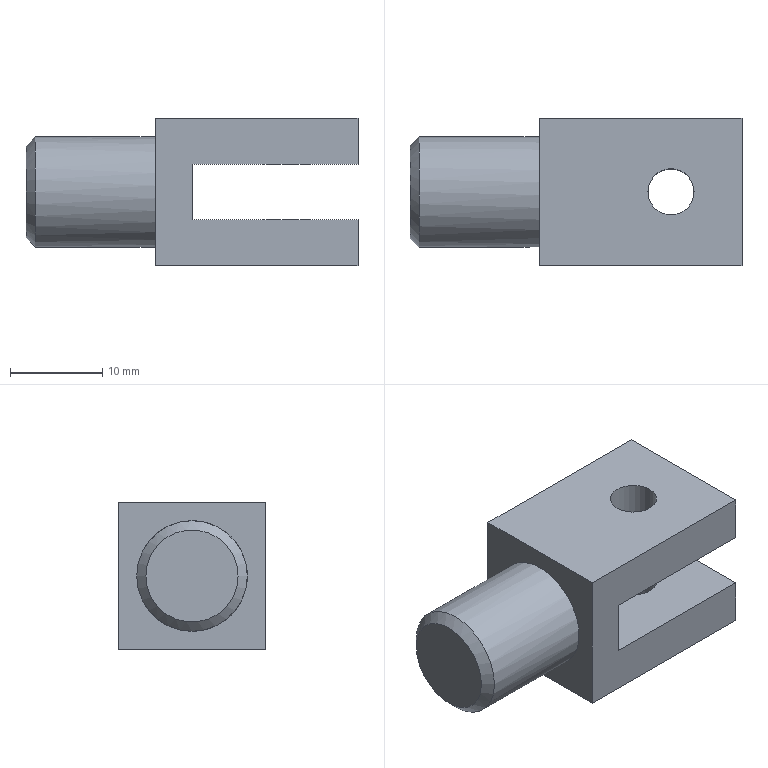Component | NX | CONNECTOR | 1 solid | 15 faces | box 36 x 16 x 16 mm | volume 5273 mm3 | plane 11 | cylinder 3 | cone 1 | commonest cylinder face diameters 5 x2 12 x1
STEP:
#1=CARTESIAN_POINT('',(0.,0.,0.));
#2=DIRECTION('',(0.,0.,1.));
#3=DIRECTION('',(1.,0.,0.));
#4=AXIS2_PLACEMENT_3D('',#1,#2,#3);
#5=CARTESIAN_POINT('',(-35.,-51.25,-19.5));
#6=VERTEX_POINT('',#5);
#7=CARTESIAN_POINT('',(-17.,-51.25,-19.5));
#8=VERTEX_POINT('',#7);
#9=CARTESIAN_POINT('',(-17.,-51.25,-19.5));
#10=DIRECTION('',(1.,0.,0.));
#11=VECTOR('',#10,1.);
#12=LINE('',#9,#11);
#13=CARTESIAN_POINT('',(-17.,-51.25,-8.5));
#14=DIRECTION('',(0.,1.,0.));
#15=DIRECTION('',(-1.,0.,0.));
#16=AXIS2_PLACEMENT_3D('',#13,#14,#15);
#17=PLANE('',#16);
#18=CARTESIAN_POINT('',(0.,-11.));
#19=DIRECTION('',(-1.,0.));
#20=VECTOR('',#19,1.);
#21=LINE('',#18,#20);
#22=(GEOMETRIC_REPRESENTATION_CONTEXT(2)PARAMETRIC_REPRESENTATION_CONTEXT()REPRESENTATION_CONTEXT('',''));
#23=DEFINITIONAL_REPRESENTATION('',(#21),#22);
#24=PCURVE('',#17,#23);
#25=CARTESIAN_POINT('',(-15.,-21.25,-19.5));
#26=DIRECTION('',(0.,0.,1.));
#27=DIRECTION('',(1.,0.,0.));
#28=AXIS2_PLACEMENT_3D('',#25,#26,#27);
#29=PLANE('',#28);
#30=CARTESIAN_POINT('',(-2.,-30.));
#31=DIRECTION('',(1.,0.));
#32=VECTOR('',#31,1.);
#33=LINE('',#30,#32);
#34=(GEOMETRIC_REPRESENTATION_CONTEXT(2)PARAMETRIC_REPRESENTATION_CONTEXT()REPRESENTATION_CONTEXT('',''));
#35=DEFINITIONAL_REPRESENTATION('',(#33),#34);
#36=PCURVE('',#29,#35);
#37=SURFACE_CURVE('',#12,(#24,#36),.PCURVE_S1.);
#38=EDGE_CURVE('',#6,#8,#37,.T.);
#39=ORIENTED_EDGE('',*,*,#38,.F.);
#40=CARTESIAN_POINT('',(-35.,-51.25,-13.5));
#41=VERTEX_POINT('',#40);
#42=CARTESIAN_POINT('',(-35.,-51.25,-8.5));
#43=DIRECTION('',(0.,0.,-1.));
#44=VECTOR('',#43,1.);
#45=LINE('',#42,#44);
#46=CARTESIAN_POINT('',(18.,0.));
#47=DIRECTION('',(0.,-1.));
#48=VECTOR('',#47,1.);
#49=LINE('',#46,#48);
#50=(GEOMETRIC_REPRESENTATION_CONTEXT(2)PARAMETRIC_REPRESENTATION_CONTEXT()REPRESENTATION_CONTEXT('',''));
#51=DEFINITIONAL_REPRESENTATION('',(#49),#50);
#52=PCURVE('',#17,#51);
#53=CARTESIAN_POINT('',(-35.,-21.25,-19.5));
#54=DIRECTION('',(1.,0.,0.));
#55=DIRECTION('',(0.,1.,0.));
#56=AXIS2_PLACEMENT_3D('',#53,#54,#55);
#57=PLANE('',#56);
#58=CARTESIAN_POINT('',(-30.,11.));
#59=DIRECTION('',(0.,-1.));
#60=VECTOR('',#59,1.);
#61=LINE('',#58,#60);
#62=(GEOMETRIC_REPRESENTATION_CONTEXT(2)PARAMETRIC_REPRESENTATION_CONTEXT()REPRESENTATION_CONTEXT('',''));
#63=DEFINITIONAL_REPRESENTATION('',(#61),#62);
#64=PCURVE('',#57,#63);
#65=SURFACE_CURVE('',#45,(#52,#64),.PCURVE_S1.);
#66=EDGE_CURVE('',#41,#6,#65,.T.);
#67=ORIENTED_EDGE('',*,*,#66,.F.);
#68=CARTESIAN_POINT('',(-17.,-51.25,-13.5));
#69=VERTEX_POINT('',#68);
#70=CARTESIAN_POINT('',(-17.,-51.25,-13.5));
#71=DIRECTION('',(-1.,0.,0.));
#72=VECTOR('',#71,1.);
#73=LINE('',#70,#72);
#74=CARTESIAN_POINT('',(0.,-5.));
#75=DIRECTION('',(1.,0.));
#76=VECTOR('',#75,1.);
#77=LINE('',#74,#76);
#78=(GEOMETRIC_REPRESENTATION_CONTEXT(2)PARAMETRIC_REPRESENTATION_CONTEXT()REPRESENTATION_CONTEXT('',''));
#79=DEFINITIONAL_REPRESENTATION('',(#77),#78);
#80=PCURVE('',#17,#79);
#81=CARTESIAN_POINT('',(-35.,-21.25,-13.5));
#82=DIRECTION('',(0.,0.,-1.));
#83=DIRECTION('',(-1.,0.,0.));
#84=AXIS2_PLACEMENT_3D('',#81,#82,#83);
#85=PLANE('',#84);
#86=CARTESIAN_POINT('',(-18.,-30.));
#87=DIRECTION('',(1.,0.));
#88=VECTOR('',#87,1.);
#89=LINE('',#86,#88);
#90=(GEOMETRIC_REPRESENTATION_CONTEXT(2)PARAMETRIC_REPRESENTATION_CONTEXT()REPRESENTATION_CONTEXT('',''));
#91=DEFINITIONAL_REPRESENTATION('',(#89),#90);
#92=PCURVE('',#85,#91);
#93=SURFACE_CURVE('',#73,(#80,#92),.PCURVE_S1.);
#94=EDGE_CURVE('',#69,#41,#93,.T.);
#95=ORIENTED_EDGE('',*,*,#94,.F.);
#96=CARTESIAN_POINT('',(-17.,-51.25,-8.5));
#97=VERTEX_POINT('',#96);
#98=CARTESIAN_POINT('',(-17.,-51.25,-8.5));
#99=DIRECTION('',(0.,0.,-1.));
#100=VECTOR('',#99,1.);
#101=LINE('',#98,#100);
#102=CARTESIAN_POINT('',(0.,0.));
#103=DIRECTION('',(0.,-1.));
#104=VECTOR('',#103,1.);
#105=LINE('',#102,#104);
#106=(GEOMETRIC_REPRESENTATION_CONTEXT(2)PARAMETRIC_REPRESENTATION_CONTEXT()REPRESENTATION_CONTEXT('',''));
#107=DEFINITIONAL_REPRESENTATION('',(#105),#106);
#108=PCURVE('',#17,#107);
#109=CARTESIAN_POINT('',(-17.,-43.25,-16.5));
#110=DIRECTION('',(1.,0.,0.));
#111=DIRECTION('',(0.,1.,0.));
#112=AXIS2_PLACEMENT_3D('',#109,#110,#111);
#113=PLANE('',#112);
#114=CARTESIAN_POINT('',(-8.,8.));
#115=DIRECTION('',(0.,-1.));
#116=VECTOR('',#115,1.);
#117=LINE('',#114,#116);
#118=(GEOMETRIC_REPRESENTATION_CONTEXT(2)PARAMETRIC_REPRESENTATION_CONTEXT()REPRESENTATION_CONTEXT('',''));
#119=DEFINITIONAL_REPRESENTATION('',(#117),#118);
#120=PCURVE('',#113,#119);
#121=SURFACE_CURVE('',#101,(#108,#120),.PCURVE_S1.);
#122=EDGE_CURVE('',#97,#69,#121,.T.);
#123=ORIENTED_EDGE('',*,*,#122,.F.);
#124=CARTESIAN_POINT('',(-39.,-51.25,-8.5));
#125=VERTEX_POINT('',#124);
#126=CARTESIAN_POINT('',(-17.,-51.25,-8.5));
#127=DIRECTION('',(-1.,0.,0.));
#128=VECTOR('',#127,1.);
#129=LINE('',#126,#128);
#130=CARTESIAN_POINT('',(0.,0.));
#131=DIRECTION('',(1.,0.));
#132=VECTOR('',#131,1.);
#133=LINE('',#130,#132);
#134=(GEOMETRIC_REPRESENTATION_CONTEXT(2)PARAMETRIC_REPRESENTATION_CONTEXT()REPRESENTATION_CONTEXT('',''));
#135=DEFINITIONAL_REPRESENTATION('',(#133),#134);
#136=PCURVE('',#17,#135);
#137=CARTESIAN_POINT('',(-17.,-35.25,-8.5));
#138=DIRECTION('',(0.,0.,-1.));
#139=DIRECTION('',(-1.,0.,0.));
#140=AXIS2_PLACEMENT_3D('',#137,#138,#139);
#141=PLANE('',#140);
#142=CARTESIAN_POINT('',(0.,-16.));
#143=DIRECTION('',(1.,0.));
#144=VECTOR('',#143,1.);
#145=LINE('',#142,#144);
#146=(GEOMETRIC_REPRESENTATION_CONTEXT(2)PARAMETRIC_REPRESENTATION_CONTEXT()REPRESENTATION_CONTEXT('',''));
#147=DEFINITIONAL_REPRESENTATION('',(#145),#146);
#148=PCURVE('',#141,#147);
#149=SURFACE_CURVE('',#129,(#136,#148),.PCURVE_S1.);
#150=EDGE_CURVE('',#97,#125,#149,.T.);
#151=ORIENTED_EDGE('',*,*,#150,.T.);
#152=CARTESIAN_POINT('',(-39.,-51.25,-24.5));
#153=VERTEX_POINT('',#152);
#154=CARTESIAN_POINT('',(-39.,-51.25,-8.5));
#155=DIRECTION('',(0.,0.,-1.));
#156=VECTOR('',#155,1.);
#157=LINE('',#154,#156);
#158=CARTESIAN_POINT('',(22.,0.));
#159=DIRECTION('',(0.,-1.));
#160=VECTOR('',#159,1.);
#161=LINE('',#158,#160);
#162=(GEOMETRIC_REPRESENTATION_CONTEXT(2)PARAMETRIC_REPRESENTATION_CONTEXT()REPRESENTATION_CONTEXT('',''));
#163=DEFINITIONAL_REPRESENTATION('',(#161),#162);
#164=PCURVE('',#17,#163);
#165=CARTESIAN_POINT('',(-39.,-43.25,-16.5));
#166=DIRECTION('',(1.,0.,0.));
#167=DIRECTION('',(0.,1.,0.));
#168=AXIS2_PLACEMENT_3D('',#165,#166,#167);
#169=PLANE('',#168);
#170=CARTESIAN_POINT('',(-8.,8.));
#171=DIRECTION('',(0.,-1.));
#172=VECTOR('',#171,1.);
#173=LINE('',#170,#172);
#174=(GEOMETRIC_REPRESENTATION_CONTEXT(2)PARAMETRIC_REPRESENTATION_CONTEXT()REPRESENTATION_CONTEXT('',''));
#175=DEFINITIONAL_REPRESENTATION('',(#173),#174);
#176=PCURVE('',#169,#175);
#177=SURFACE_CURVE('',#157,(#164,#176),.PCURVE_S1.);
#178=EDGE_CURVE('',#125,#153,#177,.T.);
#179=ORIENTED_EDGE('',*,*,#178,.T.);
#180=CARTESIAN_POINT('',(-17.,-51.25,-24.5));
#181=VERTEX_POINT('',#180);
#182=CARTESIAN_POINT('',(-17.,-51.25,-24.5));
#183=DIRECTION('',(-1.,0.,0.));
#184=VECTOR('',#183,1.);
#185=LINE('',#182,#184);
#186=CARTESIAN_POINT('',(0.,-16.));
#187=DIRECTION('',(1.,0.));
#188=VECTOR('',#187,1.);
#189=LINE('',#186,#188);
#190=(GEOMETRIC_REPRESENTATION_CONTEXT(2)PARAMETRIC_REPRESENTATION_CONTEXT()REPRESENTATION_CONTEXT('',''));
#191=DEFINITIONAL_REPRESENTATION('',(#189),#190);
#192=PCURVE('',#17,#191);
#193=CARTESIAN_POINT('',(-17.,-51.25,-24.5));
#194=DIRECTION('',(0.,0.,1.));
#195=DIRECTION('',(1.,0.,0.));
#196=AXIS2_PLACEMENT_3D('',#193,#194,#195);
#197=PLANE('',#196);
#198=CARTESIAN_POINT('',(0.,0.));
#199=DIRECTION('',(-1.,0.));
#200=VECTOR('',#199,1.);
#201=LINE('',#198,#200);
#202=(GEOMETRIC_REPRESENTATION_CONTEXT(2)PARAMETRIC_REPRESENTATION_CONTEXT()REPRESENTATION_CONTEXT('',''));
#203=DEFINITIONAL_REPRESENTATION('',(#201),#202);
#204=PCURVE('',#197,#203);
#205=SURFACE_CURVE('',#185,(#192,#204),.PCURVE_S1.);
#206=EDGE_CURVE('',#181,#153,#205,.T.);
#207=ORIENTED_EDGE('',*,*,#206,.F.);
#208=CARTESIAN_POINT('',(-17.,-51.25,-8.5));
#209=DIRECTION('',(0.,0.,-1.));
#210=VECTOR('',#209,1.);
#211=LINE('',#208,#210);
#212=CARTESIAN_POINT('',(0.,0.));
#213=DIRECTION('',(0.,-1.));
#214=VECTOR('',#213,1.);
#215=LINE('',#212,#214);
#216=(GEOMETRIC_REPRESENTATION_CONTEXT(2)PARAMETRIC_REPRESENTATION_CONTEXT()REPRESENTATION_CONTEXT('',''));
#217=DEFINITIONAL_REPRESENTATION('',(#215),#216);
#218=PCURVE('',#17,#217);
#219=CARTESIAN_POINT('',(-17.,-43.25,-16.5));
#220=DIRECTION('',(1.,0.,0.));
#221=DIRECTION('',(0.,1.,0.));
#222=AXIS2_PLACEMENT_3D('',#219,#220,#221);
#223=PLANE('',#222);
#224=CARTESIAN_POINT('',(-8.,8.));
#225=DIRECTION('',(0.,-1.));
#226=VECTOR('',#225,1.);
#227=LINE('',#224,#226);
#228=(GEOMETRIC_REPRESENTATION_CONTEXT(2)PARAMETRIC_REPRESENTATION_CONTEXT()REPRESENTATION_CONTEXT('',''));
#229=DEFINITIONAL_REPRESENTATION('',(#227),#228);
#230=PCURVE('',#223,#229);
#231=SURFACE_CURVE('',#211,(#218,#230),.PCURVE_S1.);
#232=EDGE_CURVE('',#8,#181,#231,.T.);
#233=ORIENTED_EDGE('',*,*,#232,.F.);
#234=EDGE_LOOP('',(#39,#67,#95,#123,#151,#179,#207,#233));
#235=FACE_BOUND('',#234,.T.);
#236=ADVANCED_FACE('',(#235),#17,.F.);
#237=CARTESIAN_POINT('',(-17.,-35.25,-19.5));
#238=VERTEX_POINT('',#237);
#239=CARTESIAN_POINT('',(-35.,-35.25,-19.5));
#240=VERTEX_POINT('',#239);
#241=CARTESIAN_POINT('',(-17.,-35.25,-19.5));
#242=DIRECTION('',(-1.,0.,0.));
#243=VECTOR('',#242,1.);
#244=LINE('',#241,#243);
#245=CARTESIAN_POINT('',(-17.,-35.25,-24.5));
#246=DIRECTION('',(0.,-1.,0.));
#247=DIRECTION('',(1.,0.,0.));
#248=AXIS2_PLACEMENT_3D('',#245,#246,#247);
#249=PLANE('',#248);
#250=CARTESIAN_POINT('',(0.,5.));
#251=DIRECTION('',(-1.,0.));
#252=VECTOR('',#251,1.);
#253=LINE('',#250,#252);
#254=(GEOMETRIC_REPRESENTATION_CONTEXT(2)PARAMETRIC_REPRESENTATION_CONTEXT()REPRESENTATION_CONTEXT('',''));
#255=DEFINITIONAL_REPRESENTATION('',(#253),#254);
#256=PCURVE('',#249,#255);
#257=CARTESIAN_POINT('',(-2.,-14.));
#258=DIRECTION('',(-1.,0.));
#259=VECTOR('',#258,1.);
#260=LINE('',#257,#259);
#261=(GEOMETRIC_REPRESENTATION_CONTEXT(2)PARAMETRIC_REPRESENTATION_CONTEXT()REPRESENTATION_CONTEXT('',''));
#262=DEFINITIONAL_REPRESENTATION('',(#260),#261);
#263=PCURVE('',#29,#262);
#264=SURFACE_CURVE('',#244,(#256,#263),.PCURVE_S1.);
#265=EDGE_CURVE('',#238,#240,#264,.T.);
#266=ORIENTED_EDGE('',*,*,#265,.F.);
#267=CARTESIAN_POINT('',(-17.,-35.25,-24.5));
#268=VERTEX_POINT('',#267);
#269=CARTESIAN_POINT('',(-17.,-35.25,-24.5));
#270=DIRECTION('',(0.,0.,1.));
#271=VECTOR('',#270,1.);
#272=LINE('',#269,#271);
#273=CARTESIAN_POINT('',(0.,0.));
#274=DIRECTION('',(0.,1.));
#275=VECTOR('',#274,1.);
#276=LINE('',#273,#275);
#277=(GEOMETRIC_REPRESENTATION_CONTEXT(2)PARAMETRIC_REPRESENTATION_CONTEXT()REPRESENTATION_CONTEXT('',''));
#278=DEFINITIONAL_REPRESENTATION('',(#276),#277);
#279=PCURVE('',#249,#278);
#280=CARTESIAN_POINT('',(8.,-8.));
#281=DIRECTION('',(0.,1.));
#282=VECTOR('',#281,1.);
#283=LINE('',#280,#282);
#284=(GEOMETRIC_REPRESENTATION_CONTEXT(2)PARAMETRIC_REPRESENTATION_CONTEXT()REPRESENTATION_CONTEXT('',''));
#285=DEFINITIONAL_REPRESENTATION('',(#283),#284);
#286=PCURVE('',#223,#285);
#287=SURFACE_CURVE('',#272,(#279,#286),.PCURVE_S1.);
#288=EDGE_CURVE('',#268,#238,#287,.T.);
#289=ORIENTED_EDGE('',*,*,#288,.F.);
#290=CARTESIAN_POINT('',(-39.,-35.25,-24.5));
#291=VERTEX_POINT('',#290);
#292=CARTESIAN_POINT('',(-17.,-35.25,-24.5));
#293=DIRECTION('',(-1.,0.,0.));
#294=VECTOR('',#293,1.);
#295=LINE('',#292,#294);
#296=CARTESIAN_POINT('',(0.,0.));
#297=DIRECTION('',(-1.,0.));
#298=VECTOR('',#297,1.);
#299=LINE('',#296,#298);
#300=(GEOMETRIC_REPRESENTATION_CONTEXT(2)PARAMETRIC_REPRESENTATION_CONTEXT()REPRESENTATION_CONTEXT('',''));
#301=DEFINITIONAL_REPRESENTATION('',(#299),#300);
#302=PCURVE('',#249,#301);
#303=CARTESIAN_POINT('',(0.,16.));
#304=DIRECTION('',(-1.,0.));
#305=VECTOR('',#304,1.);
#306=LINE('',#303,#305);
#307=(GEOMETRIC_REPRESENTATION_CONTEXT(2)PARAMETRIC_REPRESENTATION_CONTEXT()REPRESENTATION_CONTEXT('',''));
#308=DEFINITIONAL_REPRESENTATION('',(#306),#307);
#309=PCURVE('',#197,#308);
#310=SURFACE_CURVE('',#295,(#302,#309),.PCURVE_S1.);
#311=EDGE_CURVE('',#268,#291,#310,.T.);
#312=ORIENTED_EDGE('',*,*,#311,.T.);
#313=CARTESIAN_POINT('',(-39.,-35.25,-8.5));
#314=VERTEX_POINT('',#313);
#315=CARTESIAN_POINT('',(-39.,-35.25,-24.5));
#316=DIRECTION('',(0.,0.,1.));
#317=VECTOR('',#316,1.);
#318=LINE('',#315,#317);
#319=CARTESIAN_POINT('',(-22.,0.));
#320=DIRECTION('',(0.,1.));
#321=VECTOR('',#320,1.);
#322=LINE('',#319,#321);
#323=(GEOMETRIC_REPRESENTATION_CONTEXT(2)PARAMETRIC_REPRESENTATION_CONTEXT()REPRESENTATION_CONTEXT('',''));
#324=DEFINITIONAL_REPRESENTATION('',(#322),#323);
#325=PCURVE('',#249,#324);
#326=CARTESIAN_POINT('',(8.,-8.));
#327=DIRECTION('',(0.,1.));
#328=VECTOR('',#327,1.);
#329=LINE('',#326,#328);
#330=(GEOMETRIC_REPRESENTATION_CONTEXT(2)PARAMETRIC_REPRESENTATION_CONTEXT()REPRESENTATION_CONTEXT('',''));
#331=DEFINITIONAL_REPRESENTATION('',(#329),#330);
#332=PCURVE('',#169,#331);
#333=SURFACE_CURVE('',#318,(#325,#332),.PCURVE_S1.);
#334=EDGE_CURVE('',#291,#314,#333,.T.);
#335=ORIENTED_EDGE('',*,*,#334,.T.);
#336=CARTESIAN_POINT('',(-17.,-35.25,-8.5));
#337=VERTEX_POINT('',#336);
#338=CARTESIAN_POINT('',(-17.,-35.25,-8.5));
#339=DIRECTION('',(-1.,0.,0.));
#340=VECTOR('',#339,1.);
#341=LINE('',#338,#340);
#342=CARTESIAN_POINT('',(0.,16.));
#343=DIRECTION('',(-1.,0.));
#344=VECTOR('',#343,1.);
#345=LINE('',#342,#344);
#346=(GEOMETRIC_REPRESENTATION_CONTEXT(2)PARAMETRIC_REPRESENTATION_CONTEXT()REPRESENTATION_CONTEXT('',''));
#347=DEFINITIONAL_REPRESENTATION('',(#345),#346);
#348=PCURVE('',#249,#347);
#349=CARTESIAN_POINT('',(0.,0.));
#350=DIRECTION('',(1.,0.));
#351=VECTOR('',#350,1.);
#352=LINE('',#349,#351);
#353=(GEOMETRIC_REPRESENTATION_CONTEXT(2)PARAMETRIC_REPRESENTATION_CONTEXT()REPRESENTATION_CONTEXT('',''));
#354=DEFINITIONAL_REPRESENTATION('',(#352),#353);
#355=PCURVE('',#141,#354);
#356=SURFACE_CURVE('',#341,(#348,#355),.PCURVE_S1.);
#357=EDGE_CURVE('',#337,#314,#356,.T.);
#358=ORIENTED_EDGE('',*,*,#357,.F.);
#359=CARTESIAN_POINT('',(-17.,-35.25,-13.5));
#360=VERTEX_POINT('',#359);
#361=CARTESIAN_POINT('',(-17.,-35.25,-24.5));
#362=DIRECTION('',(0.,0.,1.));
#363=VECTOR('',#362,1.);
#364=LINE('',#361,#363);
#365=CARTESIAN_POINT('',(0.,0.));
#366=DIRECTION('',(0.,1.));
#367=VECTOR('',#366,1.);
#368=LINE('',#365,#367);
#369=(GEOMETRIC_REPRESENTATION_CONTEXT(2)PARAMETRIC_REPRESENTATION_CONTEXT()REPRESENTATION_CONTEXT('',''));
#370=DEFINITIONAL_REPRESENTATION('',(#368),#369);
#371=PCURVE('',#249,#370);
#372=CARTESIAN_POINT('',(8.,-8.));
#373=DIRECTION('',(0.,1.));
#374=VECTOR('',#373,1.);
#375=LINE('',#372,#374);
#376=(GEOMETRIC_REPRESENTATION_CONTEXT(2)PARAMETRIC_REPRESENTATION_CONTEXT()REPRESENTATION_CONTEXT('',''));
#377=DEFINITIONAL_REPRESENTATION('',(#375),#376);
#378=PCURVE('',#113,#377);
#379=SURFACE_CURVE('',#364,(#371,#378),.PCURVE_S1.);
#380=EDGE_CURVE('',#360,#337,#379,.T.);
#381=ORIENTED_EDGE('',*,*,#380,.F.);
#382=CARTESIAN_POINT('',(-35.,-35.25,-13.5));
#383=VERTEX_POINT('',#382);
#384=CARTESIAN_POINT('',(-17.,-35.25,-13.5));
#385=DIRECTION('',(1.,0.,0.));
#386=VECTOR('',#385,1.);
#387=LINE('',#384,#386);
#388=CARTESIAN_POINT('',(0.,11.));
#389=DIRECTION('',(1.,0.));
#390=VECTOR('',#389,1.);
#391=LINE('',#388,#390);
#392=(GEOMETRIC_REPRESENTATION_CONTEXT(2)PARAMETRIC_REPRESENTATION_CONTEXT()REPRESENTATION_CONTEXT('',''));
#393=DEFINITIONAL_REPRESENTATION('',(#391),#392);
#394=PCURVE('',#249,#393);
#395=CARTESIAN_POINT('',(-18.,-14.));
#396=DIRECTION('',(-1.,0.));
#397=VECTOR('',#396,1.);
#398=LINE('',#395,#397);
#399=(GEOMETRIC_REPRESENTATION_CONTEXT(2)PARAMETRIC_REPRESENTATION_CONTEXT()REPRESENTATION_CONTEXT('',''));
#400=DEFINITIONAL_REPRESENTATION('',(#398),#399);
#401=PCURVE('',#85,#400);
#402=SURFACE_CURVE('',#387,(#394,#401),.PCURVE_S1.);
#403=EDGE_CURVE('',#383,#360,#402,.T.);
#404=ORIENTED_EDGE('',*,*,#403,.F.);
#405=CARTESIAN_POINT('',(-35.,-35.25,-24.5));
#406=DIRECTION('',(0.,0.,1.));
#407=VECTOR('',#406,1.);
#408=LINE('',#405,#407);
#409=CARTESIAN_POINT('',(-18.,0.));
#410=DIRECTION('',(0.,1.));
#411=VECTOR('',#410,1.);
#412=LINE('',#409,#411);
#413=(GEOMETRIC_REPRESENTATION_CONTEXT(2)PARAMETRIC_REPRESENTATION_CONTEXT()REPRESENTATION_CONTEXT('',''));
#414=DEFINITIONAL_REPRESENTATION('',(#412),#413);
#415=PCURVE('',#249,#414);
#416=CARTESIAN_POINT('',(-14.,-5.));
#417=DIRECTION('',(0.,1.));
#418=VECTOR('',#417,1.);
#419=LINE('',#416,#418);
#420=(GEOMETRIC_REPRESENTATION_CONTEXT(2)PARAMETRIC_REPRESENTATION_CONTEXT()REPRESENTATION_CONTEXT('',''));
#421=DEFINITIONAL_REPRESENTATION('',(#419),#420);
#422=PCURVE('',#57,#421);
#423=SURFACE_CURVE('',#408,(#415,#422),.PCURVE_S1.);
#424=EDGE_CURVE('',#240,#383,#423,.T.);
#425=ORIENTED_EDGE('',*,*,#424,.F.);
#426=EDGE_LOOP('',(#266,#289,#312,#335,#358,#381,#404,#425));
#427=FACE_BOUND('',#426,.T.);
#428=ADVANCED_FACE('',(#427),#249,.F.);
#429=ORIENTED_EDGE('',*,*,#288,.T.);
#430=CARTESIAN_POINT('',(-17.,-43.25,-19.5));
#431=DIRECTION('',(0.,-1.,0.));
#432=VECTOR('',#431,1.);
#433=LINE('',#430,#432);
#434=CARTESIAN_POINT('',(0.,-3.));
#435=DIRECTION('',(-1.,0.));
#436=VECTOR('',#435,1.);
#437=LINE('',#434,#436);
#438=(GEOMETRIC_REPRESENTATION_CONTEXT(2)PARAMETRIC_REPRESENTATION_CONTEXT()REPRESENTATION_CONTEXT('',''));
#439=DEFINITIONAL_REPRESENTATION('',(#437),#438);
#440=PCURVE('',#223,#439);
#441=CARTESIAN_POINT('',(-2.,-22.));
#442=DIRECTION('',(0.,-1.));
#443=VECTOR('',#442,1.);
#444=LINE('',#441,#443);
#445=(GEOMETRIC_REPRESENTATION_CONTEXT(2)PARAMETRIC_REPRESENTATION_CONTEXT()REPRESENTATION_CONTEXT('',''));
#446=DEFINITIONAL_REPRESENTATION('',(#444),#445);
#447=PCURVE('',#29,#446);
#448=SURFACE_CURVE('',#433,(#440,#447),.PCURVE_S1.);
#449=EDGE_CURVE('',#238,#8,#448,.T.);
#450=ORIENTED_EDGE('',*,*,#449,.T.);
#451=ORIENTED_EDGE('',*,*,#232,.T.);
#452=CARTESIAN_POINT('',(-17.,-51.25,-24.5));
#453=DIRECTION('',(0.,1.,0.));
#454=VECTOR('',#453,1.);
#455=LINE('',#452,#454);
#456=CARTESIAN_POINT('',(-8.,-8.));
#457=DIRECTION('',(1.,0.));
#458=VECTOR('',#457,1.);
#459=LINE('',#456,#458);
#460=(GEOMETRIC_REPRESENTATION_CONTEXT(2)PARAMETRIC_REPRESENTATION_CONTEXT()REPRESENTATION_CONTEXT('',''));
#461=DEFINITIONAL_REPRESENTATION('',(#459),#460);
#462=PCURVE('',#223,#461);
#463=CARTESIAN_POINT('',(0.,0.));
#464=DIRECTION('',(0.,1.));
#465=VECTOR('',#464,1.);
#466=LINE('',#463,#465);
#467=(GEOMETRIC_REPRESENTATION_CONTEXT(2)PARAMETRIC_REPRESENTATION_CONTEXT()REPRESENTATION_CONTEXT('',''));
#468=DEFINITIONAL_REPRESENTATION('',(#466),#467);
#469=PCURVE('',#197,#468);
#470=SURFACE_CURVE('',#455,(#462,#469),.PCURVE_S1.);
#471=EDGE_CURVE('',#181,#268,#470,.T.);
#472=ORIENTED_EDGE('',*,*,#471,.T.);
#473=EDGE_LOOP('',(#429,#450,#451,#472));
#474=FACE_BOUND('',#473,.T.);
#475=ADVANCED_FACE('',(#474),#223,.T.);
#476=ORIENTED_EDGE('',*,*,#122,.T.);
#477=CARTESIAN_POINT('',(-17.,-43.25,-13.5));
#478=DIRECTION('',(0.,1.,0.));
#479=VECTOR('',#478,1.);
#480=LINE('',#477,#479);
#481=CARTESIAN_POINT('',(0.,3.));
#482=DIRECTION('',(1.,0.));
#483=VECTOR('',#482,1.);
#484=LINE('',#481,#483);
#485=(GEOMETRIC_REPRESENTATION_CONTEXT(2)PARAMETRIC_REPRESENTATION_CONTEXT()REPRESENTATION_CONTEXT('',''));
#486=DEFINITIONAL_REPRESENTATION('',(#484),#485);
#487=PCURVE('',#113,#486);
#488=CARTESIAN_POINT('',(-18.,-22.));
#489=DIRECTION('',(0.,1.));
#490=VECTOR('',#489,1.);
#491=LINE('',#488,#490);
#492=(GEOMETRIC_REPRESENTATION_CONTEXT(2)PARAMETRIC_REPRESENTATION_CONTEXT()REPRESENTATION_CONTEXT('',''));
#493=DEFINITIONAL_REPRESENTATION('',(#491),#492);
#494=PCURVE('',#85,#493);
#495=SURFACE_CURVE('',#480,(#487,#494),.PCURVE_S1.);
#496=EDGE_CURVE('',#69,#360,#495,.T.);
#497=ORIENTED_EDGE('',*,*,#496,.T.);
#498=ORIENTED_EDGE('',*,*,#380,.T.);
#499=CARTESIAN_POINT('',(-17.,-35.25,-8.5));
#500=DIRECTION('',(0.,-1.,0.));
#501=VECTOR('',#500,1.);
#502=LINE('',#499,#501);
#503=CARTESIAN_POINT('',(8.,8.));
#504=DIRECTION('',(-1.,0.));
#505=VECTOR('',#504,1.);
#506=LINE('',#503,#505);
#507=(GEOMETRIC_REPRESENTATION_CONTEXT(2)PARAMETRIC_REPRESENTATION_CONTEXT()REPRESENTATION_CONTEXT('',''));
#508=DEFINITIONAL_REPRESENTATION('',(#506),#507);
#509=PCURVE('',#113,#508);
#510=CARTESIAN_POINT('',(0.,0.));
#511=DIRECTION('',(0.,-1.));
#512=VECTOR('',#511,1.);
#513=LINE('',#510,#512);
#514=(GEOMETRIC_REPRESENTATION_CONTEXT(2)PARAMETRIC_REPRESENTATION_CONTEXT()REPRESENTATION_CONTEXT('',''));
#515=DEFINITIONAL_REPRESENTATION('',(#513),#514);
#516=PCURVE('',#141,#515);
#517=SURFACE_CURVE('',#502,(#509,#516),.PCURVE_S1.);
#518=EDGE_CURVE('',#337,#97,#517,.T.);
#519=ORIENTED_EDGE('',*,*,#518,.T.);
#520=EDGE_LOOP('',(#476,#497,#498,#519));
#521=FACE_BOUND('',#520,.T.);
#522=ADVANCED_FACE('',(#521),#113,.T.);
#523=CARTESIAN_POINT('',(-53.,-48.25,-16.5));
#524=VERTEX_POINT('',#523);
#525=CARTESIAN_POINT('',(-53.,-43.25,-16.5));
#526=DIRECTION('',(-1.,0.,0.));
#527=DIRECTION('',(0.,-1.,0.));
#528=AXIS2_PLACEMENT_3D('',#525,#526,#527);
#529=CIRCLE('',#528,5.);
#530=CARTESIAN_POINT('',(-53.,-43.25,-16.5));
#531=DIRECTION('',(-1.,0.,0.));
#532=DIRECTION('',(0.,-1.,0.));
#533=AXIS2_PLACEMENT_3D('',#530,#531,#532);
#534=PLANE('',#533);
#535=CARTESIAN_POINT('',(0.,0.));
#536=DIRECTION('',(1.,0.));
#537=AXIS2_PLACEMENT_2D('',#535,#536);
#538=CIRCLE('',#537,5.);
#539=(GEOMETRIC_REPRESENTATION_CONTEXT(2)PARAMETRIC_REPRESENTATION_CONTEXT()REPRESENTATION_CONTEXT('',''));
#540=DEFINITIONAL_REPRESENTATION('',(#538),#539);
#541=PCURVE('',#534,#540);
#542=CARTESIAN_POINT('',(-52.,-43.25,-16.5));
#543=DIRECTION('',(1.,0.,0.));
#544=DIRECTION('',(0.,1.,0.));
#545=AXIS2_PLACEMENT_3D('',#542,#543,#544);
#546=CONICAL_SURFACE('',#545,6.,0.7854);
#547=CARTESIAN_POINT('',(9.425,-1.));
#548=DIRECTION('',(-1.,0.));
#549=VECTOR('',#548,1.);
#550=LINE('',#547,#549);
#551=(GEOMETRIC_REPRESENTATION_CONTEXT(2)PARAMETRIC_REPRESENTATION_CONTEXT()REPRESENTATION_CONTEXT('',''));
#552=DEFINITIONAL_REPRESENTATION('',(#550),#551);
#553=PCURVE('',#546,#552);
#554=SURFACE_CURVE('',#529,(#541,#553),.PCURVE_S1.);
#555=EDGE_CURVE('',#524,#524,#554,.T.);
#556=ORIENTED_EDGE('',*,*,#555,.T.);
#557=EDGE_LOOP('',(#556));
#558=FACE_BOUND('',#557,.T.);
#559=ADVANCED_FACE('',(#558),#534,.T.);
#560=CARTESIAN_POINT('',(-52.,-49.25,-16.5));
#561=VERTEX_POINT('',#560);
#562=CARTESIAN_POINT('',(-52.,-37.25,-16.5));
#563=VERTEX_POINT('',#562);
#564=CARTESIAN_POINT('',(-52.,-43.25,-16.5));
#565=DIRECTION('',(1.,0.,0.));
#566=DIRECTION('',(0.,-1.,0.));
#567=AXIS2_PLACEMENT_3D('',#564,#565,#566);
#568=CIRCLE('',#567,6.);
#569=CARTESIAN_POINT('',(-53.,-43.25,-16.5));
#570=DIRECTION('',(1.,0.,0.));
#571=DIRECTION('',(0.,1.,0.));
#572=AXIS2_PLACEMENT_3D('',#569,#570,#571);
#573=CYLINDRICAL_SURFACE('',#572,6.);
#574=CARTESIAN_POINT('',(3.142,1.));
#575=DIRECTION('',(1.,0.));
#576=VECTOR('',#575,1.);
#577=LINE('',#574,#576);
#578=(GEOMETRIC_REPRESENTATION_CONTEXT(2)PARAMETRIC_REPRESENTATION_CONTEXT()REPRESENTATION_CONTEXT('',''));
#579=DEFINITIONAL_REPRESENTATION('',(#577),#578);
#580=PCURVE('',#573,#579);
#581=CARTESIAN_POINT('',(3.142,0.));
#582=DIRECTION('',(1.,0.));
#583=VECTOR('',#582,1.);
#584=LINE('',#581,#583);
#585=(GEOMETRIC_REPRESENTATION_CONTEXT(2)PARAMETRIC_REPRESENTATION_CONTEXT()REPRESENTATION_CONTEXT('',''));
#586=DEFINITIONAL_REPRESENTATION('',(#584),#585);
#587=PCURVE('',#546,#586);
#588=SURFACE_CURVE('',#568,(#580,#587),.PCURVE_S1.);
#589=EDGE_CURVE('',#561,#563,#588,.T.);
#590=ORIENTED_EDGE('',*,*,#589,.T.);
#591=CARTESIAN_POINT('',(-39.,-37.25,-16.5));
#592=VERTEX_POINT('',#591);
#593=CARTESIAN_POINT('',(-52.,-37.25,-16.5));
#594=CARTESIAN_POINT('',(-39.,-37.25,-16.5));
#595=B_SPLINE_CURVE_WITH_KNOTS('',1,(#593,#594),.UNSPECIFIED.,.F.,.F.,(2,2),(1.,14.),.PIECEWISE_BEZIER_KNOTS.);
#596=CARTESIAN_POINT('',(6.283,0.));
#597=DIRECTION('',(0.,1.));
#598=VECTOR('',#597,1.);
#599=LINE('',#596,#598);
#600=(GEOMETRIC_REPRESENTATION_CONTEXT(2)PARAMETRIC_REPRESENTATION_CONTEXT()REPRESENTATION_CONTEXT('',''));
#601=DEFINITIONAL_REPRESENTATION('',(#599),#600);
#602=PCURVE('',#573,#601);
#603=CARTESIAN_POINT('',(0.,0.));
#604=DIRECTION('',(0.,1.));
#605=VECTOR('',#604,1.);
#606=LINE('',#603,#605);
#607=(GEOMETRIC_REPRESENTATION_CONTEXT(2)PARAMETRIC_REPRESENTATION_CONTEXT()REPRESENTATION_CONTEXT('',''));
#608=DEFINITIONAL_REPRESENTATION('',(#606),#607);
#609=PCURVE('',#573,#608);
#610=SEAM_CURVE('',#595,(#602,#609),.PCURVE_S1.);
#611=EDGE_CURVE('',#563,#592,#610,.T.);
#612=ORIENTED_EDGE('',*,*,#611,.T.);
#613=CARTESIAN_POINT('',(-39.,-43.25,-16.5));
#614=DIRECTION('',(-1.,0.,0.));
#615=DIRECTION('',(0.,1.,0.));
#616=AXIS2_PLACEMENT_3D('',#613,#614,#615);
#617=CIRCLE('',#616,6.);
#618=CARTESIAN_POINT('',(6.283,14.));
#619=DIRECTION('',(-1.,0.));
#620=VECTOR('',#619,1.);
#621=LINE('',#618,#620);
#622=(GEOMETRIC_REPRESENTATION_CONTEXT(2)PARAMETRIC_REPRESENTATION_CONTEXT()REPRESENTATION_CONTEXT('',''));
#623=DEFINITIONAL_REPRESENTATION('',(#621),#622);
#624=PCURVE('',#573,#623);
#625=CARTESIAN_POINT('',(6.,0.));
#626=CARTESIAN_POINT('',(6.,-10.392));
#627=CARTESIAN_POINT('',(-3.,-5.196));
#628=CARTESIAN_POINT('',(-12.,-0.));
#629=CARTESIAN_POINT('',(-3.,5.196));
#630=CARTESIAN_POINT('',(6.,10.392));
#631=CARTESIAN_POINT('',(6.,0.));
#632=(BOUNDED_CURVE()B_SPLINE_CURVE(2,(#625,#626,#627,#628,#629,#630,#631),.UNSPECIFIED.,.T.,.F.)B_SPLINE_CURVE_WITH_KNOTS((1,2,2,2,2,1),(-2.094,0.,2.094,4.189,6.283,8.378),.UNSPECIFIED.)CURVE()GEOMETRIC_REPRESENTATION_ITEM()RATIONAL_B_SPLINE_CURVE((1.,0.5,1.,0.5,1.,0.5,1.))REPRESENTATION_ITEM(''));
#633=(GEOMETRIC_REPRESENTATION_CONTEXT(2)PARAMETRIC_REPRESENTATION_CONTEXT()REPRESENTATION_CONTEXT('',''));
#634=DEFINITIONAL_REPRESENTATION('',(#632),#633);
#635=PCURVE('',#169,#634);
#636=SURFACE_CURVE('',#617,(#624,#635),.PCURVE_S1.);
#637=EDGE_CURVE('',#592,#592,#636,.T.);
#638=ORIENTED_EDGE('',*,*,#637,.T.);
#639=ORIENTED_EDGE('',*,*,#611,.F.);
#640=CARTESIAN_POINT('',(-52.,-43.25,-16.5));
#641=DIRECTION('',(1.,0.,0.));
#642=DIRECTION('',(0.,-1.,0.));
#643=AXIS2_PLACEMENT_3D('',#640,#641,#642);
#644=CIRCLE('',#643,6.);
#645=CARTESIAN_POINT('',(-3.142,1.));
#646=DIRECTION('',(1.,0.));
#647=VECTOR('',#646,1.);
#648=LINE('',#645,#647);
#649=(GEOMETRIC_REPRESENTATION_CONTEXT(2)PARAMETRIC_REPRESENTATION_CONTEXT()REPRESENTATION_CONTEXT('',''));
#650=DEFINITIONAL_REPRESENTATION('',(#648),#649);
#651=PCURVE('',#573,#650);
#652=CARTESIAN_POINT('',(3.142,0.));
#653=DIRECTION('',(1.,0.));
#654=VECTOR('',#653,1.);
#655=LINE('',#652,#654);
#656=(GEOMETRIC_REPRESENTATION_CONTEXT(2)PARAMETRIC_REPRESENTATION_CONTEXT()REPRESENTATION_CONTEXT('',''));
#657=DEFINITIONAL_REPRESENTATION('',(#655),#656);
#658=PCURVE('',#546,#657);
#659=SURFACE_CURVE('',#644,(#651,#658),.PCURVE_S1.);
#660=EDGE_CURVE('',#563,#561,#659,.T.);
#661=ORIENTED_EDGE('',*,*,#660,.T.);
#662=EDGE_LOOP('',(#590,#612,#638,#639,#661));
#663=FACE_BOUND('',#662,.T.);
#664=ADVANCED_FACE('',(#663),#573,.T.);
#665=CARTESIAN_POINT('',(-22.2,-43.25,-24.5));
#666=VERTEX_POINT('',#665);
#667=CARTESIAN_POINT('',(-24.7,-43.25,-24.5));
#668=DIRECTION('',(0.,0.,-1.));
#669=DIRECTION('',(1.,0.,0.));
#670=AXIS2_PLACEMENT_3D('',#667,#668,#669);
#671=CIRCLE('',#670,2.5);
#672=CARTESIAN_POINT('',(-5.2,8.));
#673=CARTESIAN_POINT('',(-5.2,3.67));
#674=CARTESIAN_POINT('',(-8.95,5.835));
#675=CARTESIAN_POINT('',(-12.7,8.));
#676=CARTESIAN_POINT('',(-8.95,10.165));
#677=CARTESIAN_POINT('',(-5.2,12.33));
#678=CARTESIAN_POINT('',(-5.2,8.));
#679=(BOUNDED_CURVE()B_SPLINE_CURVE(2,(#672,#673,#674,#675,#676,#677,#678),.UNSPECIFIED.,.T.,.F.)B_SPLINE_CURVE_WITH_KNOTS((1,2,2,2,2,1),(-2.094,0.,2.094,4.189,6.283,8.378),.UNSPECIFIED.)CURVE()GEOMETRIC_REPRESENTATION_ITEM()RATIONAL_B_SPLINE_CURVE((1.,0.5,1.,0.5,1.,0.5,1.))REPRESENTATION_ITEM(''));
#680=(GEOMETRIC_REPRESENTATION_CONTEXT(2)PARAMETRIC_REPRESENTATION_CONTEXT()REPRESENTATION_CONTEXT('',''));
#681=DEFINITIONAL_REPRESENTATION('',(#679),#680);
#682=PCURVE('',#197,#681);
#683=CARTESIAN_POINT('',(-24.7,-43.25,-38.5));
#684=DIRECTION('',(0.,0.,1.));
#685=DIRECTION('',(1.,0.,0.));
#686=AXIS2_PLACEMENT_3D('',#683,#684,#685);
#687=CYLINDRICAL_SURFACE('',#686,2.5);
#688=CARTESIAN_POINT('',(6.283,14.));
#689=DIRECTION('',(-1.,0.));
#690=VECTOR('',#689,1.);
#691=LINE('',#688,#690);
#692=(GEOMETRIC_REPRESENTATION_CONTEXT(2)PARAMETRIC_REPRESENTATION_CONTEXT()REPRESENTATION_CONTEXT('',''));
#693=DEFINITIONAL_REPRESENTATION('',(#691),#692);
#694=PCURVE('',#687,#693);
#695=SURFACE_CURVE('',#671,(#682,#694),.PCURVE_S1.);
#696=EDGE_CURVE('',#666,#666,#695,.T.);
#697=ORIENTED_EDGE('',*,*,#696,.F.);
#698=EDGE_LOOP('',(#697));
#699=FACE_BOUND('',#698,.T.);
#700=CARTESIAN_POINT('',(-39.,-51.25,-24.5));
#701=DIRECTION('',(0.,1.,0.));
#702=VECTOR('',#701,1.);
#703=LINE('',#700,#702);
#704=CARTESIAN_POINT('',(-22.,0.));
#705=DIRECTION('',(0.,1.));
#706=VECTOR('',#705,1.);
#707=LINE('',#704,#706);
#708=(GEOMETRIC_REPRESENTATION_CONTEXT(2)PARAMETRIC_REPRESENTATION_CONTEXT()REPRESENTATION_CONTEXT('',''));
#709=DEFINITIONAL_REPRESENTATION('',(#707),#708);
#710=PCURVE('',#197,#709);
#711=CARTESIAN_POINT('',(-8.,-8.));
#712=DIRECTION('',(1.,0.));
#713=VECTOR('',#712,1.);
#714=LINE('',#711,#713);
#715=(GEOMETRIC_REPRESENTATION_CONTEXT(2)PARAMETRIC_REPRESENTATION_CONTEXT()REPRESENTATION_CONTEXT('',''));
#716=DEFINITIONAL_REPRESENTATION('',(#714),#715);
#717=PCURVE('',#169,#716);
#718=SURFACE_CURVE('',#703,(#710,#717),.PCURVE_S1.);
#719=EDGE_CURVE('',#153,#291,#718,.T.);
#720=ORIENTED_EDGE('',*,*,#719,.T.);
#721=ORIENTED_EDGE('',*,*,#311,.F.);
#722=ORIENTED_EDGE('',*,*,#471,.F.);
#723=ORIENTED_EDGE('',*,*,#206,.T.);
#724=EDGE_LOOP('',(#720,#721,#722,#723));
#725=FACE_BOUND('',#724,.T.);
#726=ADVANCED_FACE('',(#699,#725),#197,.F.);
#727=CARTESIAN_POINT('',(-27.2,-43.25,-8.5));
#728=VERTEX_POINT('',#727);
#729=CARTESIAN_POINT('',(-24.7,-43.25,-8.5));
#730=DIRECTION('',(0.,0.,1.));
#731=DIRECTION('',(-1.,0.,0.));
#732=AXIS2_PLACEMENT_3D('',#729,#730,#731);
#733=CIRCLE('',#732,2.5);
#734=CARTESIAN_POINT('',(10.2,-8.));
#735=CARTESIAN_POINT('',(10.2,-12.33));
#736=CARTESIAN_POINT('',(6.45,-10.165));
#737=CARTESIAN_POINT('',(2.7,-8.));
#738=CARTESIAN_POINT('',(6.45,-5.835));
#739=CARTESIAN_POINT('',(10.2,-3.67));
#740=CARTESIAN_POINT('',(10.2,-8.));
#741=(BOUNDED_CURVE()B_SPLINE_CURVE(2,(#734,#735,#736,#737,#738,#739,#740),.UNSPECIFIED.,.T.,.F.)B_SPLINE_CURVE_WITH_KNOTS((1,2,2,2,2,1),(-2.094,0.,2.094,4.189,6.283,8.378),.UNSPECIFIED.)CURVE()GEOMETRIC_REPRESENTATION_ITEM()RATIONAL_B_SPLINE_CURVE((1.,0.5,1.,0.5,1.,0.5,1.))REPRESENTATION_ITEM(''));
#742=(GEOMETRIC_REPRESENTATION_CONTEXT(2)PARAMETRIC_REPRESENTATION_CONTEXT()REPRESENTATION_CONTEXT('',''));
#743=DEFINITIONAL_REPRESENTATION('',(#741),#742);
#744=PCURVE('',#141,#743);
#745=CARTESIAN_POINT('',(-24.7,-43.25,-38.5));
#746=DIRECTION('',(0.,0.,1.));
#747=DIRECTION('',(1.,0.,0.));
#748=AXIS2_PLACEMENT_3D('',#745,#746,#747);
#749=CYLINDRICAL_SURFACE('',#748,2.5);
#750=CARTESIAN_POINT('',(3.142,30.));
#751=DIRECTION('',(1.,0.));
#752=VECTOR('',#751,1.);
#753=LINE('',#750,#752);
#754=(GEOMETRIC_REPRESENTATION_CONTEXT(2)PARAMETRIC_REPRESENTATION_CONTEXT()REPRESENTATION_CONTEXT('',''));
#755=DEFINITIONAL_REPRESENTATION('',(#753),#754);
#756=PCURVE('',#749,#755);
#757=SURFACE_CURVE('',#733,(#744,#756),.PCURVE_S1.);
#758=EDGE_CURVE('',#728,#728,#757,.T.);
#759=ORIENTED_EDGE('',*,*,#758,.F.);
#760=EDGE_LOOP('',(#759));
#761=FACE_BOUND('',#760,.T.);
#762=CARTESIAN_POINT('',(-39.,-35.25,-8.5));
#763=DIRECTION('',(0.,-1.,0.));
#764=VECTOR('',#763,1.);
#765=LINE('',#762,#764);
#766=CARTESIAN_POINT('',(22.,0.));
#767=DIRECTION('',(0.,-1.));
#768=VECTOR('',#767,1.);
#769=LINE('',#766,#768);
#770=(GEOMETRIC_REPRESENTATION_CONTEXT(2)PARAMETRIC_REPRESENTATION_CONTEXT()REPRESENTATION_CONTEXT('',''));
#771=DEFINITIONAL_REPRESENTATION('',(#769),#770);
#772=PCURVE('',#141,#771);
#773=CARTESIAN_POINT('',(8.,8.));
#774=DIRECTION('',(-1.,0.));
#775=VECTOR('',#774,1.);
#776=LINE('',#773,#775);
#777=(GEOMETRIC_REPRESENTATION_CONTEXT(2)PARAMETRIC_REPRESENTATION_CONTEXT()REPRESENTATION_CONTEXT('',''));
#778=DEFINITIONAL_REPRESENTATION('',(#776),#777);
#779=PCURVE('',#169,#778);
#780=SURFACE_CURVE('',#765,(#772,#779),.PCURVE_S1.);
#781=EDGE_CURVE('',#314,#125,#780,.T.);
#782=ORIENTED_EDGE('',*,*,#781,.T.);
#783=ORIENTED_EDGE('',*,*,#150,.F.);
#784=ORIENTED_EDGE('',*,*,#518,.F.);
#785=ORIENTED_EDGE('',*,*,#357,.T.);
#786=EDGE_LOOP('',(#782,#783,#784,#785));
#787=FACE_BOUND('',#786,.T.);
#788=ADVANCED_FACE('',(#761,#787),#141,.F.);
#789=ORIENTED_EDGE('',*,*,#637,.F.);
#790=EDGE_LOOP('',(#789));
#791=FACE_BOUND('',#790,.T.);
#792=ORIENTED_EDGE('',*,*,#178,.F.);
#793=ORIENTED_EDGE('',*,*,#781,.F.);
#794=ORIENTED_EDGE('',*,*,#334,.F.);
#795=ORIENTED_EDGE('',*,*,#719,.F.);
#796=EDGE_LOOP('',(#792,#793,#794,#795));
#797=FACE_BOUND('',#796,.T.);
#798=ADVANCED_FACE('',(#791,#797),#169,.F.);
#799=ORIENTED_EDGE('',*,*,#66,.T.);
#800=CARTESIAN_POINT('',(-35.,-21.25,-19.5));
#801=DIRECTION('',(0.,1.,0.));
#802=VECTOR('',#801,1.);
#803=LINE('',#800,#802);
#804=CARTESIAN_POINT('',(0.,0.));
#805=DIRECTION('',(1.,0.));
#806=VECTOR('',#805,1.);
#807=LINE('',#804,#806);
#808=(GEOMETRIC_REPRESENTATION_CONTEXT(2)PARAMETRIC_REPRESENTATION_CONTEXT()REPRESENTATION_CONTEXT('',''));
#809=DEFINITIONAL_REPRESENTATION('',(#807),#808);
#810=PCURVE('',#57,#809);
#811=CARTESIAN_POINT('',(-20.,0.));
#812=DIRECTION('',(0.,1.));
#813=VECTOR('',#812,1.);
#814=LINE('',#811,#813);
#815=(GEOMETRIC_REPRESENTATION_CONTEXT(2)PARAMETRIC_REPRESENTATION_CONTEXT()REPRESENTATION_CONTEXT('',''));
#816=DEFINITIONAL_REPRESENTATION('',(#814),#815);
#817=PCURVE('',#29,#816);
#818=SURFACE_CURVE('',#803,(#810,#817),.PCURVE_S1.);
#819=EDGE_CURVE('',#6,#240,#818,.T.);
#820=ORIENTED_EDGE('',*,*,#819,.T.);
#821=ORIENTED_EDGE('',*,*,#424,.T.);
#822=CARTESIAN_POINT('',(-35.,-21.25,-13.5));
#823=DIRECTION('',(0.,1.,0.));
#824=VECTOR('',#823,1.);
#825=LINE('',#822,#824);
#826=CARTESIAN_POINT('',(0.,6.));
#827=DIRECTION('',(1.,0.));
#828=VECTOR('',#827,1.);
#829=LINE('',#826,#828);
#830=(GEOMETRIC_REPRESENTATION_CONTEXT(2)PARAMETRIC_REPRESENTATION_CONTEXT()REPRESENTATION_CONTEXT('',''));
#831=DEFINITIONAL_REPRESENTATION('',(#829),#830);
#832=PCURVE('',#57,#831);
#833=CARTESIAN_POINT('',(0.,0.));
#834=DIRECTION('',(0.,1.));
#835=VECTOR('',#834,1.);
#836=LINE('',#833,#835);
#837=(GEOMETRIC_REPRESENTATION_CONTEXT(2)PARAMETRIC_REPRESENTATION_CONTEXT()REPRESENTATION_CONTEXT('',''));
#838=DEFINITIONAL_REPRESENTATION('',(#836),#837);
#839=PCURVE('',#85,#838);
#840=SURFACE_CURVE('',#825,(#832,#839),.PCURVE_S1.);
#841=EDGE_CURVE('',#41,#383,#840,.T.);
#842=ORIENTED_EDGE('',*,*,#841,.F.);
#843=EDGE_LOOP('',(#799,#820,#821,#842));
#844=FACE_BOUND('',#843,.T.);
#845=ADVANCED_FACE('',(#844),#57,.T.);
#846=CARTESIAN_POINT('',(-22.2,-43.25,-19.5));
#847=VERTEX_POINT('',#846);
#848=CARTESIAN_POINT('',(-24.7,-43.25,-19.5));
#849=DIRECTION('',(0.,0.,-1.));
#850=DIRECTION('',(1.,0.,0.));
#851=AXIS2_PLACEMENT_3D('',#848,#849,#850);
#852=CIRCLE('',#851,2.5);
#853=CARTESIAN_POINT('',(-7.2,-22.));
#854=CARTESIAN_POINT('',(-7.2,-26.33));
#855=CARTESIAN_POINT('',(-10.95,-24.165));
#856=CARTESIAN_POINT('',(-14.7,-22.));
#857=CARTESIAN_POINT('',(-10.95,-19.835));
#858=CARTESIAN_POINT('',(-7.2,-17.67));
#859=CARTESIAN_POINT('',(-7.2,-22.));
#860=(BOUNDED_CURVE()B_SPLINE_CURVE(2,(#853,#854,#855,#856,#857,#858,#859),.UNSPECIFIED.,.T.,.F.)B_SPLINE_CURVE_WITH_KNOTS((1,2,2,2,2,1),(-2.094,0.,2.094,4.189,6.283,8.378),.UNSPECIFIED.)CURVE()GEOMETRIC_REPRESENTATION_ITEM()RATIONAL_B_SPLINE_CURVE((1.,0.5,1.,0.5,1.,0.5,1.))REPRESENTATION_ITEM(''));
#861=(GEOMETRIC_REPRESENTATION_CONTEXT(2)PARAMETRIC_REPRESENTATION_CONTEXT()REPRESENTATION_CONTEXT('',''));
#862=DEFINITIONAL_REPRESENTATION('',(#860),#861);
#863=PCURVE('',#29,#862);
#864=CARTESIAN_POINT('',(6.283,19.));
#865=DIRECTION('',(-1.,0.));
#866=VECTOR('',#865,1.);
#867=LINE('',#864,#866);
#868=(GEOMETRIC_REPRESENTATION_CONTEXT(2)PARAMETRIC_REPRESENTATION_CONTEXT()REPRESENTATION_CONTEXT('',''));
#869=DEFINITIONAL_REPRESENTATION('',(#867),#868);
#870=PCURVE('',#687,#869);
#871=SURFACE_CURVE('',#852,(#863,#870),.PCURVE_S1.);
#872=EDGE_CURVE('',#847,#847,#871,.T.);
#873=ORIENTED_EDGE('',*,*,#872,.T.);
#874=EDGE_LOOP('',(#873));
#875=FACE_BOUND('',#874,.T.);
#876=ORIENTED_EDGE('',*,*,#38,.T.);
#877=ORIENTED_EDGE('',*,*,#449,.F.);
#878=ORIENTED_EDGE('',*,*,#265,.T.);
#879=ORIENTED_EDGE('',*,*,#819,.F.);
#880=EDGE_LOOP('',(#876,#877,#878,#879));
#881=FACE_BOUND('',#880,.T.);
#882=ADVANCED_FACE('',(#875,#881),#29,.T.);
#883=CARTESIAN_POINT('',(-27.2,-43.25,-13.5));
#884=VERTEX_POINT('',#883);
#885=CARTESIAN_POINT('',(-24.7,-43.25,-13.5));
#886=DIRECTION('',(0.,0.,1.));
#887=DIRECTION('',(-1.,0.,0.));
#888=AXIS2_PLACEMENT_3D('',#885,#886,#887);
#889=CIRCLE('',#888,2.5);
#890=CARTESIAN_POINT('',(-7.8,-22.));
#891=CARTESIAN_POINT('',(-7.8,-26.33));
#892=CARTESIAN_POINT('',(-11.55,-24.165));
#893=CARTESIAN_POINT('',(-15.3,-22.));
#894=CARTESIAN_POINT('',(-11.55,-19.835));
#895=CARTESIAN_POINT('',(-7.8,-17.67));
#896=CARTESIAN_POINT('',(-7.8,-22.));
#897=(BOUNDED_CURVE()B_SPLINE_CURVE(2,(#890,#891,#892,#893,#894,#895,#896),.UNSPECIFIED.,.T.,.F.)B_SPLINE_CURVE_WITH_KNOTS((1,2,2,2,2,1),(-2.094,0.,2.094,4.189,6.283,8.378),.UNSPECIFIED.)CURVE()GEOMETRIC_REPRESENTATION_ITEM()RATIONAL_B_SPLINE_CURVE((1.,0.5,1.,0.5,1.,0.5,1.))REPRESENTATION_ITEM(''));
#898=(GEOMETRIC_REPRESENTATION_CONTEXT(2)PARAMETRIC_REPRESENTATION_CONTEXT()REPRESENTATION_CONTEXT('',''));
#899=DEFINITIONAL_REPRESENTATION('',(#897),#898);
#900=PCURVE('',#85,#899);
#901=CARTESIAN_POINT('',(3.142,25.));
#902=DIRECTION('',(1.,0.));
#903=VECTOR('',#902,1.);
#904=LINE('',#901,#903);
#905=(GEOMETRIC_REPRESENTATION_CONTEXT(2)PARAMETRIC_REPRESENTATION_CONTEXT()REPRESENTATION_CONTEXT('',''));
#906=DEFINITIONAL_REPRESENTATION('',(#904),#905);
#907=PCURVE('',#749,#906);
#908=SURFACE_CURVE('',#889,(#900,#907),.PCURVE_S1.);
#909=EDGE_CURVE('',#884,#884,#908,.T.);
#910=ORIENTED_EDGE('',*,*,#909,.T.);
#911=EDGE_LOOP('',(#910));
#912=FACE_BOUND('',#911,.T.);
#913=ORIENTED_EDGE('',*,*,#94,.T.);
#914=ORIENTED_EDGE('',*,*,#841,.T.);
#915=ORIENTED_EDGE('',*,*,#403,.T.);
#916=ORIENTED_EDGE('',*,*,#496,.F.);
#917=EDGE_LOOP('',(#913,#914,#915,#916));
#918=FACE_BOUND('',#917,.T.);
#919=ADVANCED_FACE('',(#912,#918),#85,.T.);
#920=ORIENTED_EDGE('',*,*,#909,.T.);
#921=CARTESIAN_POINT('',(-27.2,-43.25,-13.5));
#922=CARTESIAN_POINT('',(-27.2,-43.25,-8.5));
#923=B_SPLINE_CURVE_WITH_KNOTS('',1,(#921,#922),.UNSPECIFIED.,.F.,.F.,(2,2),(25.,30.),.PIECEWISE_BEZIER_KNOTS.);
#924=CARTESIAN_POINT('',(9.425,0.));
#925=DIRECTION('',(0.,1.));
#926=VECTOR('',#925,1.);
#927=LINE('',#924,#926);
#928=(GEOMETRIC_REPRESENTATION_CONTEXT(2)PARAMETRIC_REPRESENTATION_CONTEXT()REPRESENTATION_CONTEXT('',''));
#929=DEFINITIONAL_REPRESENTATION('',(#927),#928);
#930=PCURVE('',#749,#929);
#931=CARTESIAN_POINT('',(3.142,0.));
#932=DIRECTION('',(0.,1.));
#933=VECTOR('',#932,1.);
#934=LINE('',#931,#933);
#935=(GEOMETRIC_REPRESENTATION_CONTEXT(2)PARAMETRIC_REPRESENTATION_CONTEXT()REPRESENTATION_CONTEXT('',''));
#936=DEFINITIONAL_REPRESENTATION('',(#934),#935);
#937=PCURVE('',#749,#936);
#938=SEAM_CURVE('',#923,(#930,#937),.PCURVE_S1.);
#939=EDGE_CURVE('',#884,#728,#938,.T.);
#940=ORIENTED_EDGE('',*,*,#939,.T.);
#941=ORIENTED_EDGE('',*,*,#758,.F.);
#942=ORIENTED_EDGE('',*,*,#939,.F.);
#943=EDGE_LOOP('',(#920,#940,#941,#942));
#944=FACE_BOUND('',#943,.F.);
#945=ADVANCED_FACE('',(#944),#749,.F.);
#946=ORIENTED_EDGE('',*,*,#872,.T.);
#947=CARTESIAN_POINT('',(-22.2,-43.25,-24.5));
#948=CARTESIAN_POINT('',(-22.2,-43.25,-19.5));
#949=B_SPLINE_CURVE_WITH_KNOTS('',1,(#947,#948),.UNSPECIFIED.,.F.,.F.,(2,2),(14.,19.),.PIECEWISE_BEZIER_KNOTS.);
#950=CARTESIAN_POINT('',(0.,0.));
#951=DIRECTION('',(0.,1.));
#952=VECTOR('',#951,1.);
#953=LINE('',#950,#952);
#954=(GEOMETRIC_REPRESENTATION_CONTEXT(2)PARAMETRIC_REPRESENTATION_CONTEXT()REPRESENTATION_CONTEXT('',''));
#955=DEFINITIONAL_REPRESENTATION('',(#953),#954);
#956=PCURVE('',#687,#955);
#957=CARTESIAN_POINT('',(6.283,0.));
#958=DIRECTION('',(0.,1.));
#959=VECTOR('',#958,1.);
#960=LINE('',#957,#959);
#961=(GEOMETRIC_REPRESENTATION_CONTEXT(2)PARAMETRIC_REPRESENTATION_CONTEXT()REPRESENTATION_CONTEXT('',''));
#962=DEFINITIONAL_REPRESENTATION('',(#960),#961);
#963=PCURVE('',#687,#962);
#964=SEAM_CURVE('',#949,(#956,#963),.PCURVE_S1.);
#965=EDGE_CURVE('',#666,#847,#964,.T.);
#966=ORIENTED_EDGE('',*,*,#965,.F.);
#967=ORIENTED_EDGE('',*,*,#696,.F.);
#968=ORIENTED_EDGE('',*,*,#965,.T.);
#969=EDGE_LOOP('',(#946,#966,#967,#968));
#970=FACE_BOUND('',#969,.F.);
#971=ADVANCED_FACE('',(#970),#687,.F.);
#972=ORIENTED_EDGE('',*,*,#555,.F.);
#973=CARTESIAN_POINT('',(-53.,-48.25,-16.5));
#974=CARTESIAN_POINT('',(-52.,-49.25,-16.5));
#975=B_SPLINE_CURVE_WITH_KNOTS('',1,(#973,#974),.UNSPECIFIED.,.F.,.F.,(2,2),(-1.414,0.),.PIECEWISE_BEZIER_KNOTS.);
#976=CARTESIAN_POINT('',(9.425,0.));
#977=DIRECTION('',(0.,1.));
#978=VECTOR('',#977,1.);
#979=LINE('',#976,#978);
#980=(GEOMETRIC_REPRESENTATION_CONTEXT(2)PARAMETRIC_REPRESENTATION_CONTEXT()REPRESENTATION_CONTEXT('',''));
#981=DEFINITIONAL_REPRESENTATION('',(#979),#980);
#982=PCURVE('',#546,#981);
#983=CARTESIAN_POINT('',(3.142,0.));
#984=DIRECTION('',(0.,1.));
#985=VECTOR('',#984,1.);
#986=LINE('',#983,#985);
#987=(GEOMETRIC_REPRESENTATION_CONTEXT(2)PARAMETRIC_REPRESENTATION_CONTEXT()REPRESENTATION_CONTEXT('',''));
#988=DEFINITIONAL_REPRESENTATION('',(#986),#987);
#989=PCURVE('',#546,#988);
#990=SEAM_CURVE('',#975,(#982,#989),.PCURVE_S1.);
#991=EDGE_CURVE('',#524,#561,#990,.T.);
#992=ORIENTED_EDGE('',*,*,#991,.T.);
#993=ORIENTED_EDGE('',*,*,#660,.F.);
#994=ORIENTED_EDGE('',*,*,#589,.F.);
#995=ORIENTED_EDGE('',*,*,#991,.F.);
#996=EDGE_LOOP('',(#972,#992,#993,#994,#995));
#997=FACE_BOUND('',#996,.T.);
#998=ADVANCED_FACE('',(#997),#546,.T.);
#999=CLOSED_SHELL('',(#236,#428,#475,#522,#559,#664,#726,#788,#798,#845,#882,#919,#945,#971,#998));
#1000=MANIFOLD_SOLID_BREP('',#999);
#1001=(LENGTH_UNIT()NAMED_UNIT(*)SI_UNIT(.MILLI.,.METRE.));
#1002=UNCERTAINTY_MEASURE_WITH_UNIT(LENGTH_MEASURE(0.000002),#1001,'','');
#1003=(NAMED_UNIT(*)PLANE_ANGLE_UNIT()SI_UNIT($,.RADIAN.));
#1004=(NAMED_UNIT(*)SI_UNIT($,.STERADIAN.)SOLID_ANGLE_UNIT());
#1005=(GEOMETRIC_REPRESENTATION_CONTEXT(3)GLOBAL_UNCERTAINTY_ASSIGNED_CONTEXT((#1002))GLOBAL_UNIT_ASSIGNED_CONTEXT((#1001,#1003,#1004))REPRESENTATION_CONTEXT('',''));
#1006=ADVANCED_BREP_SHAPE_REPRESENTATION('',(#4,#1000),#1005);